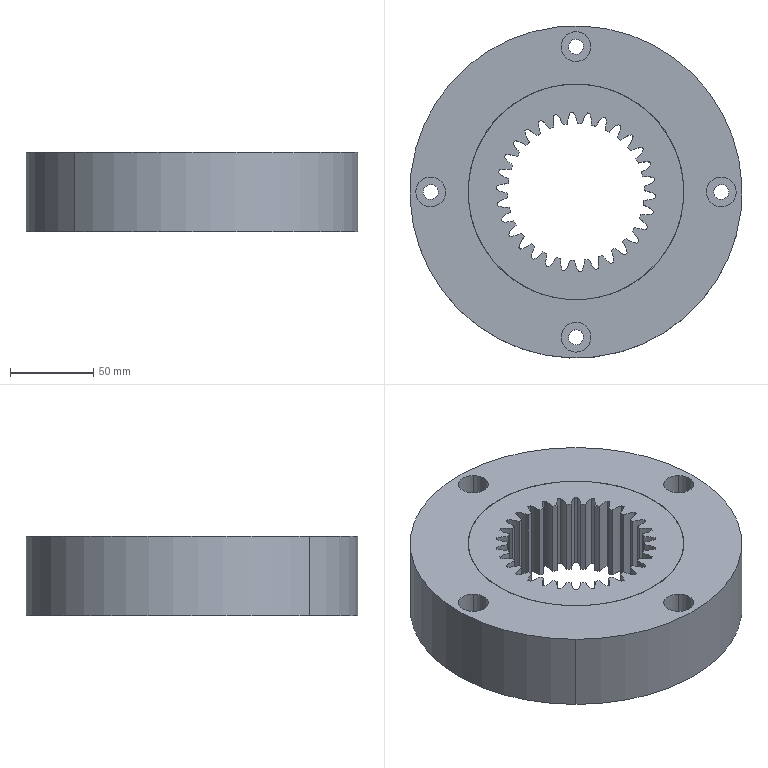Component | SolidWorks | 3-1 | 2 solids | 155 faces | volume 1185715 mm3 | cylinder 143 | plane 8 | cone 4 | commonest cylinder face diameters 36 x64 96 x31 82.498 x30 18 x8 9 x8 200 x2